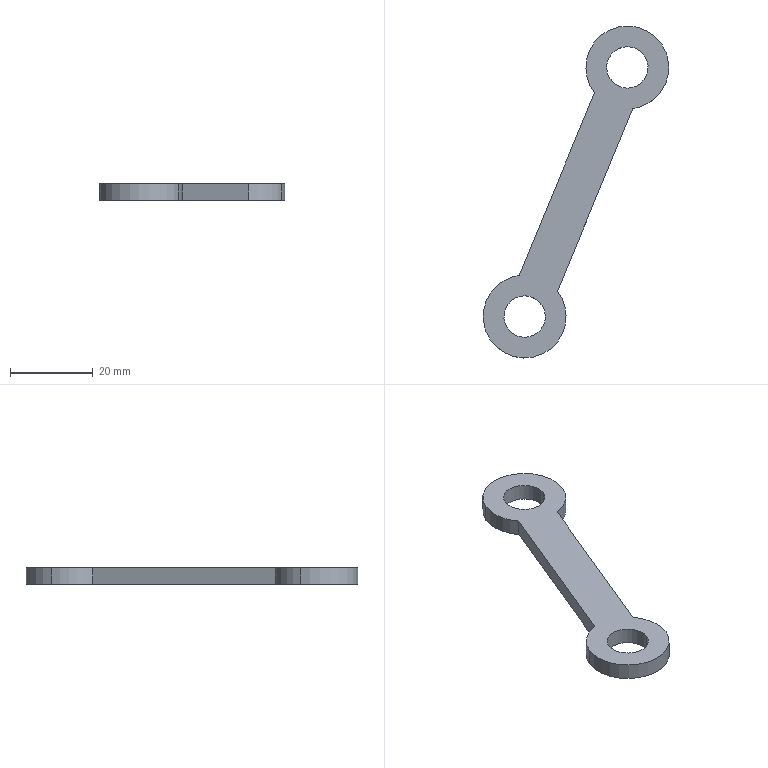Component | SolidWorks | SwingArm-1 | 1 solid | 14 faces | box 44.79 x 80.09 x 4 mm | volume 3720 mm3 | cylinder 10 | plane 4 | commonest cylinder face diameters 20 x6 10 x4
build123d program:
from build123d import *

# Parameters (mm, degrees)
SKETCH1_R           = 5
BOSS_EXTRUDE1_DEPTH = 4


with BuildPart() as part:
    # Sketch1 → Boss-Extrude1 (new body)
    with BuildSketch(Plane.XY):
        with BuildLine():
            Line((5, 26.285), (5, -21.395))
            ThreePointArc((5, -21.395), (0, -40.055), (-5, -21.395))
            Line((-5, -21.395), (-5, 26.285))
            ThreePointArc((-5, 26.285), (0, 44.945), (5, 26.285))
        make_face()
        with Locations((0, 34.945)):
            Circle(SKETCH1_R, mode=Mode.SUBTRACT)
        with Locations((0, -30.055)):
            Circle(SKETCH1_R, mode=Mode.SUBTRACT)
    extrude(amount=BOSS_EXTRUDE1_DEPTH)


solid = part.part

# Placed as in the assembly
solid = solid.moved(Location((34.398, 21.301, 108.846), (0, 0, 157.58)))
STEP:
#1=COLOUR_RGB('',0.7922,0.8196,0.9333);
#2=FILL_AREA_STYLE_COLOUR('',#1);
#3=FILL_AREA_STYLE('',(#2));
#4=SURFACE_STYLE_FILL_AREA(#3);
#5=SURFACE_SIDE_STYLE('',(#4));
#6=SURFACE_STYLE_USAGE(.BOTH.,#5);
#7=PRESENTATION_STYLE_ASSIGNMENT((#6));
#8=CARTESIAN_POINT('',(0.6476,-0.3581,4.443));
#9=VERTEX_POINT('',#8);
#10=CARTESIAN_POINT('',(1.011,-0.5083,4.443));
#11=VERTEX_POINT('',#10);
#12=CARTESIAN_POINT('',(0.8295,-0.4332,4.443));
#13=DIRECTION('',(-0.,0.,1.));
#14=DIRECTION('',(0.9244,-0.3814,0.));
#15=AXIS2_PLACEMENT_3D('',#12,#13,#14);
#16=CIRCLE('',#15,0.1969);
#17=EDGE_CURVE('',#9,#11,#16,.T.);
#18=ORIENTED_EDGE('',*,*,#17,.T.);
#19=CARTESIAN_POINT('',(1.011,-0.5083,4.285));
#20=VERTEX_POINT('',#19);
#21=CARTESIAN_POINT('',(1.011,-0.5083,4.443));
#22=DIRECTION('',(0.,-0.,-1.));
#23=VECTOR('',#22,39.37);
#24=LINE('',#21,#23);
#25=EDGE_CURVE('',#11,#20,#24,.T.);
#26=ORIENTED_EDGE('',*,*,#25,.T.);
#27=CARTESIAN_POINT('',(0.6476,-0.3581,4.285));
#28=VERTEX_POINT('',#27);
#29=CARTESIAN_POINT('',(0.8295,-0.4332,4.285));
#30=DIRECTION('',(-0.,0.,1.));
#31=DIRECTION('',(0.9244,-0.3814,0.));
#32=AXIS2_PLACEMENT_3D('',#29,#30,#31);
#33=CIRCLE('',#32,0.1969);
#34=EDGE_CURVE('',#28,#20,#33,.T.);
#35=ORIENTED_EDGE('',*,*,#34,.F.);
#36=CARTESIAN_POINT('',(0.6476,-0.3581,4.443));
#37=DIRECTION('',(0.,-0.,-1.));
#38=VECTOR('',#37,39.37);
#39=LINE('',#36,#38);
#40=EDGE_CURVE('',#9,#28,#39,.T.);
#41=ORIENTED_EDGE('',*,*,#40,.F.);
#42=EDGE_LOOP('',(#18,#26,#35,#41));
#43=FACE_OUTER_BOUND('',#42,.T.);
#44=CARTESIAN_POINT('',(0.8295,-0.4332,4.443));
#45=DIRECTION('',(0.,-0.,-1.));
#46=DIRECTION('',(-0.9244,0.3814,0.));
#47=AXIS2_PLACEMENT_3D('',#44,#45,#46);
#48=CYLINDRICAL_SURFACE('',#47,0.1969);
#49=ADVANCED_FACE('',(#43),#48,.F.);
#50=CARTESIAN_POINT('',(1.624,2.008,4.443));
#51=VERTEX_POINT('',#50);
#52=CARTESIAN_POINT('',(1.988,1.857,4.443));
#53=VERTEX_POINT('',#52);
#54=CARTESIAN_POINT('',(1.806,1.932,4.443));
#55=DIRECTION('',(-0.,0.,1.));
#56=DIRECTION('',(0.9244,-0.3814,0.));
#57=AXIS2_PLACEMENT_3D('',#54,#55,#56);
#58=CIRCLE('',#57,0.1969);
#59=EDGE_CURVE('',#51,#53,#58,.T.);
#60=ORIENTED_EDGE('',*,*,#59,.T.);
#61=CARTESIAN_POINT('',(1.988,1.857,4.285));
#62=VERTEX_POINT('',#61);
#63=CARTESIAN_POINT('',(1.988,1.857,4.443));
#64=DIRECTION('',(0.,-0.,-1.));
#65=VECTOR('',#64,39.37);
#66=LINE('',#63,#65);
#67=EDGE_CURVE('',#53,#62,#66,.T.);
#68=ORIENTED_EDGE('',*,*,#67,.T.);
#69=CARTESIAN_POINT('',(1.624,2.008,4.285));
#70=VERTEX_POINT('',#69);
#71=CARTESIAN_POINT('',(1.806,1.932,4.285));
#72=DIRECTION('',(-0.,0.,1.));
#73=DIRECTION('',(0.9244,-0.3814,0.));
#74=AXIS2_PLACEMENT_3D('',#71,#72,#73);
#75=CIRCLE('',#74,0.1969);
#76=EDGE_CURVE('',#70,#62,#75,.T.);
#77=ORIENTED_EDGE('',*,*,#76,.F.);
#78=CARTESIAN_POINT('',(1.624,2.008,4.443));
#79=DIRECTION('',(0.,-0.,-1.));
#80=VECTOR('',#79,39.37);
#81=LINE('',#78,#80);
#82=EDGE_CURVE('',#51,#70,#81,.T.);
#83=ORIENTED_EDGE('',*,*,#82,.F.);
#84=EDGE_LOOP('',(#60,#68,#77,#83));
#85=FACE_OUTER_BOUND('',#84,.T.);
#86=CARTESIAN_POINT('',(1.806,1.932,4.443));
#87=DIRECTION('',(0.,-0.,-1.));
#88=DIRECTION('',(-0.9244,0.3814,0.));
#89=AXIS2_PLACEMENT_3D('',#86,#87,#88);
#90=CYLINDRICAL_SURFACE('',#89,0.1969);
#91=ADVANCED_FACE('',(#85),#90,.F.);
#92=CARTESIAN_POINT('',(2.169,1.782,4.443));
#93=VERTEX_POINT('',#92);
#94=CARTESIAN_POINT('',(1.442,2.083,4.443));
#95=VERTEX_POINT('',#94);
#96=CARTESIAN_POINT('',(1.806,1.932,4.443));
#97=DIRECTION('',(-0.,0.,1.));
#98=DIRECTION('',(0.9244,-0.3814,0.));
#99=AXIS2_PLACEMENT_3D('',#96,#97,#98);
#100=CIRCLE('',#99,0.3937);
#101=EDGE_CURVE('',#93,#95,#100,.T.);
#102=ORIENTED_EDGE('',*,*,#101,.F.);
#103=CARTESIAN_POINT('',(2.169,1.782,4.285));
#104=VERTEX_POINT('',#103);
#105=CARTESIAN_POINT('',(2.169,1.782,4.443));
#106=DIRECTION('',(0.,-0.,-1.));
#107=VECTOR('',#106,39.37);
#108=LINE('',#105,#107);
#109=EDGE_CURVE('',#93,#104,#108,.T.);
#110=ORIENTED_EDGE('',*,*,#109,.T.);
#111=CARTESIAN_POINT('',(1.442,2.083,4.285));
#112=VERTEX_POINT('',#111);
#113=CARTESIAN_POINT('',(1.806,1.932,4.285));
#114=DIRECTION('',(-0.,0.,1.));
#115=DIRECTION('',(0.9244,-0.3814,0.));
#116=AXIS2_PLACEMENT_3D('',#113,#114,#115);
#117=CIRCLE('',#116,0.3937);
#118=EDGE_CURVE('',#104,#112,#117,.T.);
#119=ORIENTED_EDGE('',*,*,#118,.T.);
#120=CARTESIAN_POINT('',(1.442,2.083,4.443));
#121=DIRECTION('',(0.,-0.,-1.));
#122=VECTOR('',#121,39.37);
#123=LINE('',#120,#122);
#124=EDGE_CURVE('',#95,#112,#123,.T.);
#125=ORIENTED_EDGE('',*,*,#124,.F.);
#126=EDGE_LOOP('',(#102,#110,#119,#125));
#127=FACE_OUTER_BOUND('',#126,.T.);
#128=CARTESIAN_POINT('',(1.806,1.932,4.443));
#129=DIRECTION('',(0.,-0.,-1.));
#130=DIRECTION('',(-0.9244,0.3814,0.));
#131=AXIS2_PLACEMENT_3D('',#128,#129,#130);
#132=CYLINDRICAL_SURFACE('',#131,0.3937);
#133=ADVANCED_FACE('',(#127),#132,.T.);
#134=CARTESIAN_POINT('',(1.494,1.692,4.443));
#135=VERTEX_POINT('',#134);
#136=CARTESIAN_POINT('',(1.806,1.932,4.443));
#137=DIRECTION('',(-0.,0.,1.));
#138=DIRECTION('',(0.9244,-0.3814,0.));
#139=AXIS2_PLACEMENT_3D('',#136,#137,#138);
#140=CIRCLE('',#139,0.3937);
#141=EDGE_CURVE('',#95,#135,#140,.T.);
#142=ORIENTED_EDGE('',*,*,#141,.F.);
#143=ORIENTED_EDGE('',*,*,#124,.T.);
#144=CARTESIAN_POINT('',(1.494,1.692,4.285));
#145=VERTEX_POINT('',#144);
#146=CARTESIAN_POINT('',(1.806,1.932,4.285));
#147=DIRECTION('',(-0.,0.,1.));
#148=DIRECTION('',(0.9244,-0.3814,0.));
#149=AXIS2_PLACEMENT_3D('',#146,#147,#148);
#150=CIRCLE('',#149,0.3937);
#151=EDGE_CURVE('',#112,#145,#150,.T.);
#152=ORIENTED_EDGE('',*,*,#151,.T.);
#153=CARTESIAN_POINT('',(1.494,1.692,4.443));
#154=DIRECTION('',(0.,-0.,-1.));
#155=VECTOR('',#154,39.37);
#156=LINE('',#153,#155);
#157=EDGE_CURVE('',#135,#145,#156,.T.);
#158=ORIENTED_EDGE('',*,*,#157,.F.);
#159=EDGE_LOOP('',(#142,#143,#152,#158));
#160=FACE_OUTER_BOUND('',#159,.T.);
#161=CARTESIAN_POINT('',(1.806,1.932,4.443));
#162=DIRECTION('',(0.,-0.,-1.));
#163=DIRECTION('',(-0.9244,0.3814,0.));
#164=AXIS2_PLACEMENT_3D('',#161,#162,#163);
#165=CYLINDRICAL_SURFACE('',#164,0.3937);
#166=ADVANCED_FACE('',(#160),#165,.T.);
#167=CARTESIAN_POINT('',(1.193,-0.5833,4.443));
#168=VERTEX_POINT('',#167);
#169=CARTESIAN_POINT('',(1.142,-0.1931,4.443));
#170=VERTEX_POINT('',#169);
#171=CARTESIAN_POINT('',(0.8295,-0.4332,4.443));
#172=DIRECTION('',(-0.,0.,1.));
#173=DIRECTION('',(0.9244,-0.3814,0.));
#174=AXIS2_PLACEMENT_3D('',#171,#172,#173);
#175=CIRCLE('',#174,0.3937);
#176=EDGE_CURVE('',#168,#170,#175,.T.);
#177=ORIENTED_EDGE('',*,*,#176,.F.);
#178=CARTESIAN_POINT('',(1.193,-0.5833,4.285));
#179=VERTEX_POINT('',#178);
#180=CARTESIAN_POINT('',(1.193,-0.5833,4.443));
#181=DIRECTION('',(0.,-0.,-1.));
#182=VECTOR('',#181,39.37);
#183=LINE('',#180,#182);
#184=EDGE_CURVE('',#168,#179,#183,.T.);
#185=ORIENTED_EDGE('',*,*,#184,.T.);
#186=CARTESIAN_POINT('',(1.142,-0.1931,4.285));
#187=VERTEX_POINT('',#186);
#188=CARTESIAN_POINT('',(0.8295,-0.4332,4.285));
#189=DIRECTION('',(-0.,0.,1.));
#190=DIRECTION('',(0.9244,-0.3814,0.));
#191=AXIS2_PLACEMENT_3D('',#188,#189,#190);
#192=CIRCLE('',#191,0.3937);
#193=EDGE_CURVE('',#179,#187,#192,.T.);
#194=ORIENTED_EDGE('',*,*,#193,.T.);
#195=CARTESIAN_POINT('',(1.142,-0.1931,4.443));
#196=DIRECTION('',(0.,-0.,-1.));
#197=VECTOR('',#196,39.37);
#198=LINE('',#195,#197);
#199=EDGE_CURVE('',#170,#187,#198,.T.);
#200=ORIENTED_EDGE('',*,*,#199,.F.);
#201=EDGE_LOOP('',(#177,#185,#194,#200));
#202=FACE_OUTER_BOUND('',#201,.T.);
#203=CARTESIAN_POINT('',(0.8295,-0.4332,4.443));
#204=DIRECTION('',(0.,-0.,-1.));
#205=DIRECTION('',(-0.9244,0.3814,0.));
#206=AXIS2_PLACEMENT_3D('',#203,#204,#205);
#207=CYLINDRICAL_SURFACE('',#206,0.3937);
#208=ADVANCED_FACE('',(#202),#207,.T.);
#209=ORIENTED_EDGE('',*,*,#184,.F.);
#210=CARTESIAN_POINT('',(0.4656,-0.283,4.443));
#211=VERTEX_POINT('',#210);
#212=CARTESIAN_POINT('',(0.8295,-0.4332,4.443));
#213=DIRECTION('',(-0.,0.,1.));
#214=DIRECTION('',(0.9244,-0.3814,0.));
#215=AXIS2_PLACEMENT_3D('',#212,#213,#214);
#216=CIRCLE('',#215,0.3937);
#217=EDGE_CURVE('',#211,#168,#216,.T.);
#218=ORIENTED_EDGE('',*,*,#217,.F.);
#219=CARTESIAN_POINT('',(0.4656,-0.283,4.285));
#220=VERTEX_POINT('',#219);
#221=CARTESIAN_POINT('',(0.4656,-0.283,4.443));
#222=DIRECTION('',(0.,-0.,-1.));
#223=VECTOR('',#222,39.37);
#224=LINE('',#221,#223);
#225=EDGE_CURVE('',#211,#220,#224,.T.);
#226=ORIENTED_EDGE('',*,*,#225,.T.);
#227=CARTESIAN_POINT('',(0.8295,-0.4332,4.285));
#228=DIRECTION('',(-0.,0.,1.));
#229=DIRECTION('',(0.9244,-0.3814,0.));
#230=AXIS2_PLACEMENT_3D('',#227,#228,#229);
#231=CIRCLE('',#230,0.3937);
#232=EDGE_CURVE('',#220,#179,#231,.T.);
#233=ORIENTED_EDGE('',*,*,#232,.T.);
#234=EDGE_LOOP('',(#209,#218,#226,#233));
#235=FACE_OUTER_BOUND('',#234,.T.);
#236=CARTESIAN_POINT('',(0.8295,-0.4332,4.443));
#237=DIRECTION('',(0.,-0.,-1.));
#238=DIRECTION('',(-0.9244,0.3814,0.));
#239=AXIS2_PLACEMENT_3D('',#236,#237,#238);
#240=CYLINDRICAL_SURFACE('',#239,0.3937);
#241=ADVANCED_FACE('',(#235),#240,.T.);
#242=ORIENTED_EDGE('',*,*,#59,.F.);
#243=CARTESIAN_POINT('',(1.806,1.932,4.443));
#244=DIRECTION('',(-0.,0.,1.));
#245=DIRECTION('',(0.9244,-0.3814,0.));
#246=AXIS2_PLACEMENT_3D('',#243,#244,#245);
#247=CIRCLE('',#246,0.1969);
#248=EDGE_CURVE('',#53,#51,#247,.T.);
#249=ORIENTED_EDGE('',*,*,#248,.F.);
#250=EDGE_LOOP('',(#242,#249));
#251=FACE_BOUND('',#250,.T.);
#252=CARTESIAN_POINT('',(0.7776,-0.04292,4.443));
#253=VERTEX_POINT('',#252);
#254=CARTESIAN_POINT('',(0.8295,-0.4332,4.443));
#255=DIRECTION('',(-0.,0.,1.));
#256=DIRECTION('',(0.9244,-0.3814,0.));
#257=AXIS2_PLACEMENT_3D('',#254,#255,#256);
#258=CIRCLE('',#257,0.3937);
#259=EDGE_CURVE('',#253,#211,#258,.T.);
#260=ORIENTED_EDGE('',*,*,#259,.T.);
#261=ORIENTED_EDGE('',*,*,#217,.T.);
#262=ORIENTED_EDGE('',*,*,#176,.T.);
#263=CARTESIAN_POINT('',(1.857,1.542,4.443));
#264=VERTEX_POINT('',#263);
#265=CARTESIAN_POINT('',(1.857,1.542,4.443));
#266=DIRECTION('',(0.3814,0.9244,-0.));
#267=VECTOR('',#266,39.37);
#268=LINE('',#265,#267);
#269=EDGE_CURVE('',#170,#264,#268,.T.);
#270=ORIENTED_EDGE('',*,*,#269,.T.);
#271=CARTESIAN_POINT('',(1.806,1.932,4.443));
#272=DIRECTION('',(-0.,0.,1.));
#273=DIRECTION('',(0.9244,-0.3814,0.));
#274=AXIS2_PLACEMENT_3D('',#271,#272,#273);
#275=CIRCLE('',#274,0.3937);
#276=EDGE_CURVE('',#264,#93,#275,.T.);
#277=ORIENTED_EDGE('',*,*,#276,.T.);
#278=ORIENTED_EDGE('',*,*,#101,.T.);
#279=ORIENTED_EDGE('',*,*,#141,.T.);
#280=CARTESIAN_POINT('',(1.494,1.692,4.443));
#281=DIRECTION('',(-0.3814,-0.9244,0.));
#282=VECTOR('',#281,39.37);
#283=LINE('',#280,#282);
#284=EDGE_CURVE('',#135,#253,#283,.T.);
#285=ORIENTED_EDGE('',*,*,#284,.T.);
#286=EDGE_LOOP('',(#260,#261,#262,#270,#277,#278,#279,#285));
#287=FACE_OUTER_BOUND('',#286,.T.);
#288=ORIENTED_EDGE('',*,*,#17,.F.);
#289=CARTESIAN_POINT('',(0.8295,-0.4332,4.443));
#290=DIRECTION('',(-0.,0.,1.));
#291=DIRECTION('',(0.9244,-0.3814,0.));
#292=AXIS2_PLACEMENT_3D('',#289,#290,#291);
#293=CIRCLE('',#292,0.1969);
#294=EDGE_CURVE('',#11,#9,#293,.T.);
#295=ORIENTED_EDGE('',*,*,#294,.F.);
#296=EDGE_LOOP('',(#288,#295));
#297=FACE_BOUND('',#296,.T.);
#298=CARTESIAN_POINT('',(0.8295,-0.4332,4.443));
#299=DIRECTION('',(-0.,0.,1.));
#300=DIRECTION('',(0.9244,-0.3814,0.));
#301=AXIS2_PLACEMENT_3D('',#298,#299,#300);
#302=PLANE('',#301);
#303=ADVANCED_FACE('',(#251,#287,#297),#302,.T.);
#304=CARTESIAN_POINT('',(0.7776,-0.04292,4.285));
#305=VERTEX_POINT('',#304);
#306=CARTESIAN_POINT('',(0.8295,-0.4332,4.285));
#307=DIRECTION('',(-0.,0.,1.));
#308=DIRECTION('',(0.9244,-0.3814,0.));
#309=AXIS2_PLACEMENT_3D('',#306,#307,#308);
#310=CIRCLE('',#309,0.3937);
#311=EDGE_CURVE('',#305,#220,#310,.T.);
#312=ORIENTED_EDGE('',*,*,#311,.F.);
#313=CARTESIAN_POINT('',(1.494,1.692,4.285));
#314=DIRECTION('',(-0.3814,-0.9244,0.));
#315=VECTOR('',#314,39.37);
#316=LINE('',#313,#315);
#317=EDGE_CURVE('',#145,#305,#316,.T.);
#318=ORIENTED_EDGE('',*,*,#317,.F.);
#319=ORIENTED_EDGE('',*,*,#151,.F.);
#320=ORIENTED_EDGE('',*,*,#118,.F.);
#321=CARTESIAN_POINT('',(1.857,1.542,4.285));
#322=VERTEX_POINT('',#321);
#323=CARTESIAN_POINT('',(1.806,1.932,4.285));
#324=DIRECTION('',(-0.,0.,1.));
#325=DIRECTION('',(0.9244,-0.3814,0.));
#326=AXIS2_PLACEMENT_3D('',#323,#324,#325);
#327=CIRCLE('',#326,0.3937);
#328=EDGE_CURVE('',#322,#104,#327,.T.);
#329=ORIENTED_EDGE('',*,*,#328,.F.);
#330=CARTESIAN_POINT('',(1.857,1.542,4.285));
#331=DIRECTION('',(0.3814,0.9244,-0.));
#332=VECTOR('',#331,39.37);
#333=LINE('',#330,#332);
#334=EDGE_CURVE('',#187,#322,#333,.T.);
#335=ORIENTED_EDGE('',*,*,#334,.F.);
#336=ORIENTED_EDGE('',*,*,#193,.F.);
#337=ORIENTED_EDGE('',*,*,#232,.F.);
#338=EDGE_LOOP('',(#312,#318,#319,#320,#329,#335,#336,#337));
#339=FACE_OUTER_BOUND('',#338,.T.);
#340=ORIENTED_EDGE('',*,*,#76,.T.);
#341=CARTESIAN_POINT('',(1.806,1.932,4.285));
#342=DIRECTION('',(-0.,0.,1.));
#343=DIRECTION('',(0.9244,-0.3814,0.));
#344=AXIS2_PLACEMENT_3D('',#341,#342,#343);
#345=CIRCLE('',#344,0.1969);
#346=EDGE_CURVE('',#62,#70,#345,.T.);
#347=ORIENTED_EDGE('',*,*,#346,.T.);
#348=EDGE_LOOP('',(#340,#347));
#349=FACE_BOUND('',#348,.T.);
#350=ORIENTED_EDGE('',*,*,#34,.T.);
#351=CARTESIAN_POINT('',(0.8295,-0.4332,4.285));
#352=DIRECTION('',(-0.,0.,1.));
#353=DIRECTION('',(0.9244,-0.3814,0.));
#354=AXIS2_PLACEMENT_3D('',#351,#352,#353);
#355=CIRCLE('',#354,0.1969);
#356=EDGE_CURVE('',#20,#28,#355,.T.);
#357=ORIENTED_EDGE('',*,*,#356,.T.);
#358=EDGE_LOOP('',(#350,#357));
#359=FACE_BOUND('',#358,.T.);
#360=CARTESIAN_POINT('',(0.8295,-0.4332,4.285));
#361=DIRECTION('',(-0.,0.,1.));
#362=DIRECTION('',(0.9244,-0.3814,0.));
#363=AXIS2_PLACEMENT_3D('',#360,#361,#362);
#364=PLANE('',#363);
#365=ADVANCED_FACE('',(#339,#349,#359),#364,.F.);
#366=ORIENTED_EDGE('',*,*,#225,.F.);
#367=ORIENTED_EDGE('',*,*,#259,.F.);
#368=CARTESIAN_POINT('',(0.7776,-0.04292,4.443));
#369=DIRECTION('',(0.,-0.,-1.));
#370=VECTOR('',#369,39.37);
#371=LINE('',#368,#370);
#372=EDGE_CURVE('',#253,#305,#371,.T.);
#373=ORIENTED_EDGE('',*,*,#372,.T.);
#374=ORIENTED_EDGE('',*,*,#311,.T.);
#375=EDGE_LOOP('',(#366,#367,#373,#374));
#376=FACE_OUTER_BOUND('',#375,.T.);
#377=CARTESIAN_POINT('',(0.8295,-0.4332,4.443));
#378=DIRECTION('',(0.,-0.,-1.));
#379=DIRECTION('',(-0.9244,0.3814,0.));
#380=AXIS2_PLACEMENT_3D('',#377,#378,#379);
#381=CYLINDRICAL_SURFACE('',#380,0.3937);
#382=ADVANCED_FACE('',(#376),#381,.T.);
#383=ORIENTED_EDGE('',*,*,#334,.T.);
#384=CARTESIAN_POINT('',(1.857,1.542,4.443));
#385=DIRECTION('',(0.,-0.,-1.));
#386=VECTOR('',#385,39.37);
#387=LINE('',#384,#386);
#388=EDGE_CURVE('',#264,#322,#387,.T.);
#389=ORIENTED_EDGE('',*,*,#388,.F.);
#390=ORIENTED_EDGE('',*,*,#269,.F.);
#391=ORIENTED_EDGE('',*,*,#199,.T.);
#392=EDGE_LOOP('',(#383,#389,#390,#391));
#393=FACE_OUTER_BOUND('',#392,.T.);
#394=CARTESIAN_POINT('',(1.857,1.542,4.443));
#395=DIRECTION('',(-0.9244,0.3814,-0.));
#396=DIRECTION('',(-0.,0.,1.));
#397=AXIS2_PLACEMENT_3D('',#394,#395,#396);
#398=PLANE('',#397);
#399=ADVANCED_FACE('',(#393),#398,.F.);
#400=ORIENTED_EDGE('',*,*,#109,.F.);
#401=ORIENTED_EDGE('',*,*,#276,.F.);
#402=ORIENTED_EDGE('',*,*,#388,.T.);
#403=ORIENTED_EDGE('',*,*,#328,.T.);
#404=EDGE_LOOP('',(#400,#401,#402,#403));
#405=FACE_OUTER_BOUND('',#404,.T.);
#406=CARTESIAN_POINT('',(1.806,1.932,4.443));
#407=DIRECTION('',(0.,-0.,-1.));
#408=DIRECTION('',(-0.9244,0.3814,0.));
#409=AXIS2_PLACEMENT_3D('',#406,#407,#408);
#410=CYLINDRICAL_SURFACE('',#409,0.3937);
#411=ADVANCED_FACE('',(#405),#410,.T.);
#412=ORIENTED_EDGE('',*,*,#317,.T.);
#413=ORIENTED_EDGE('',*,*,#372,.F.);
#414=ORIENTED_EDGE('',*,*,#284,.F.);
#415=ORIENTED_EDGE('',*,*,#157,.T.);
#416=EDGE_LOOP('',(#412,#413,#414,#415));
#417=FACE_OUTER_BOUND('',#416,.T.);
#418=CARTESIAN_POINT('',(1.494,1.692,4.443));
#419=DIRECTION('',(0.9244,-0.3814,0.));
#420=DIRECTION('',(0.,-0.,-1.));
#421=AXIS2_PLACEMENT_3D('',#418,#419,#420);
#422=PLANE('',#421);
#423=ADVANCED_FACE('',(#417),#422,.F.);
#424=ORIENTED_EDGE('',*,*,#67,.F.);
#425=ORIENTED_EDGE('',*,*,#248,.T.);
#426=ORIENTED_EDGE('',*,*,#82,.T.);
#427=ORIENTED_EDGE('',*,*,#346,.F.);
#428=EDGE_LOOP('',(#424,#425,#426,#427));
#429=FACE_OUTER_BOUND('',#428,.T.);
#430=CARTESIAN_POINT('',(1.806,1.932,4.443));
#431=DIRECTION('',(0.,-0.,-1.));
#432=DIRECTION('',(-0.9244,0.3814,0.));
#433=AXIS2_PLACEMENT_3D('',#430,#431,#432);
#434=CYLINDRICAL_SURFACE('',#433,0.1969);
#435=ADVANCED_FACE('',(#429),#434,.F.);
#436=ORIENTED_EDGE('',*,*,#25,.F.);
#437=ORIENTED_EDGE('',*,*,#294,.T.);
#438=ORIENTED_EDGE('',*,*,#40,.T.);
#439=ORIENTED_EDGE('',*,*,#356,.F.);
#440=EDGE_LOOP('',(#436,#437,#438,#439));
#441=FACE_OUTER_BOUND('',#440,.T.);
#442=CARTESIAN_POINT('',(0.8295,-0.4332,4.443));
#443=DIRECTION('',(0.,-0.,-1.));
#444=DIRECTION('',(-0.9244,0.3814,0.));
#445=AXIS2_PLACEMENT_3D('',#442,#443,#444);
#446=CYLINDRICAL_SURFACE('',#445,0.1969);
#447=ADVANCED_FACE('',(#441),#446,.F.);
#448=CLOSED_SHELL('',(#49,#91,#133,#166,#208,#241,#303,#365,#382,#399,#411,#423,#435,#447));
#449=MANIFOLD_SOLID_BREP('',#448);
#450=STYLED_ITEM('',(#7),#449);
#451=PRESENTATION_LAYER_ASSIGNMENT('','',(#450));
#452=(LENGTH_UNIT()NAMED_UNIT(*)SI_UNIT($,.METRE.));
#453=LENGTH_MEASURE_WITH_UNIT(LENGTH_MEASURE(0.0254),#452);
#454=DIMENSIONAL_EXPONENTS(1.,0.,0.,0.,0.,0.,0.);
#455=(CONVERSION_BASED_UNIT('',#453)LENGTH_UNIT()NAMED_UNIT(#454));
#456=UNCERTAINTY_MEASURE_WITH_UNIT(LENGTH_MEASURE(0.00001),#455,'','');
#457=(NAMED_UNIT(*)PLANE_ANGLE_UNIT()SI_UNIT($,.RADIAN.));
#458=(NAMED_UNIT(*)SI_UNIT($,.STERADIAN.)SOLID_ANGLE_UNIT());
#459=(GEOMETRIC_REPRESENTATION_CONTEXT(3)GLOBAL_UNCERTAINTY_ASSIGNED_CONTEXT((#456))GLOBAL_UNIT_ASSIGNED_CONTEXT((#455,#457,#458))REPRESENTATION_CONTEXT('',''));
#460=MECHANICAL_DESIGN_GEOMETRIC_PRESENTATION_REPRESENTATION('',(#450),#459);
#461=CARTESIAN_POINT('',(0.,0.,0.));
#462=DIRECTION('',(0.,0.,1.));
#463=DIRECTION('',(1.,0.,0.));
#464=AXIS2_PLACEMENT_3D('',#461,#462,#463);
#465=(LENGTH_UNIT()NAMED_UNIT(*)SI_UNIT($,.METRE.));
#466=LENGTH_MEASURE_WITH_UNIT(LENGTH_MEASURE(0.0254),#465);
#467=DIMENSIONAL_EXPONENTS(1.,0.,0.,0.,0.,0.,0.);
#468=(CONVERSION_BASED_UNIT('',#466)LENGTH_UNIT()NAMED_UNIT(#467));
#469=UNCERTAINTY_MEASURE_WITH_UNIT(LENGTH_MEASURE(0.00001),#468,'','');
#470=(NAMED_UNIT(*)PLANE_ANGLE_UNIT()SI_UNIT($,.RADIAN.));
#471=(NAMED_UNIT(*)SI_UNIT($,.STERADIAN.)SOLID_ANGLE_UNIT());
#472=(GEOMETRIC_REPRESENTATION_CONTEXT(3)GLOBAL_UNCERTAINTY_ASSIGNED_CONTEXT((#469))GLOBAL_UNIT_ASSIGNED_CONTEXT((#468,#470,#471))REPRESENTATION_CONTEXT('',''));
#473=ADVANCED_BREP_SHAPE_REPRESENTATION('',(#449,#464),#472);